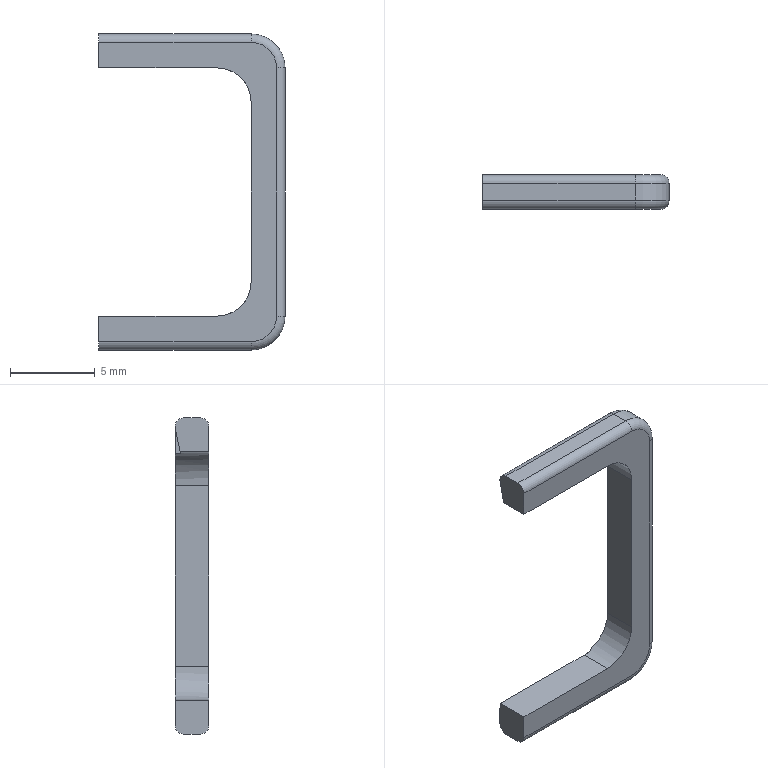Component | SolidWorks | BrushHolder-1 | 1 solid | 30 faces | box 10.95 x 2 x 18.6 mm | volume 140 mm3 | plane 16 | cylinder 10 | torus 4 | commonest cylinder face diameters 1 x6 4 x4
build123d program:
from build123d import *

# Parameters (mm, degrees)
EXTRUDE_THIN1_DEPTH           = 2
FILLET1_R                     = 2
FILLET2_R                     = 0.5
SCOOP_BENDING_CLEARANCE_DEPTH = 7.5


with BuildPart() as part:
    # Sketch1 → Extrude-Thin1 (new body)
    with BuildSketch(Plane.XY):
        Polygon((0, 0), (0, 8.954), (14.597, 8.954), (14.597, 0), (16.597, 0), (16.597, 10.954), (-2, 10.954), (-2, 0), align=None)
    extrude(amount=EXTRUDE_THIN1_DEPTH)

    # Fillet1
    fillet1_edges = [part.edges().sort_by_distance(p)[0] for p in [
        (-2, 10.954, 1),
        (16.597, 10.954, 1),
        (14.597, 8.954, 1),
        (0, 8.954, 1),
    ]]
    fillet(fillet1_edges, radius=FILLET1_R)

    # Fillet2
    fillet2_edges = [part.edges().sort_by_distance(p)[0] for p in [
        (16.597, 4.477, 2),
        (7.298, 10.954, 0),
        (7.298, 10.954, 2),
        (-2, 4.477, 0),
        (-1.414, 10.369, 0),
        (16.011, 10.369, 0),
        (-2, 4.477, 2),
        (-1.414, 10.369, 2),
        (16.011, 10.369, 2),
        (16.597, 4.477, 0),
    ]]
    fillet(fillet2_edges, radius=FILLET2_R)

    # Spatula Clearance Sketch → Scoop Bending Clearance (cut)
    with BuildSketch(Plane.XZ):
        Polygon((-1.456, 0), (0, 0.3), (0.2439, 0.3), (0.2439, -0.2446), (-1.456, -0.2446), align=None)
        Polygon((14.974, 0), (14.597, 0.04539), (14.344, 0.04539), (14.344, -0.2446), (14.974, -0.2446), align=None)
    extrude(amount=-SCOOP_BENDING_CLEARANCE_DEPTH, mode=Mode.SUBTRACT)


solid = part.part

# Placed as in the assembly
solid = solid.moved(Location((-35.654, -76.145, 205.244), (90, 0, -90)))
STEP:
#1=COLOUR_RGB('',0.7922,0.8196,0.9333);
#2=FILL_AREA_STYLE_COLOUR('',#1);
#3=FILL_AREA_STYLE('',(#2));
#4=SURFACE_STYLE_FILL_AREA(#3);
#5=SURFACE_SIDE_STYLE('',(#4));
#6=SURFACE_STYLE_USAGE(.BOTH.,#5);
#7=PRESENTATION_STYLE_ASSIGNMENT((#6));
#8=CARTESIAN_POINT('',(-1.051,-3.057,8.159));
#9=VERTEX_POINT('',#8);
#10=CARTESIAN_POINT('',(-1.051,-3.018,8.159));
#11=VERTEX_POINT('',#10);
#12=CARTESIAN_POINT('',(-1.051,-3.077,8.159));
#13=DIRECTION('',(-0.,1.,-0.));
#14=VECTOR('',#13,39.37);
#15=LINE('',#12,#14);
#16=EDGE_CURVE('',#9,#11,#15,.T.);
#17=ORIENTED_EDGE('',*,*,#16,.T.);
#18=CARTESIAN_POINT('',(-1.404,-3.018,8.159));
#19=VERTEX_POINT('',#18);
#20=CARTESIAN_POINT('',(-1.404,-3.018,8.159));
#21=DIRECTION('',(-1.,-0.,-0.));
#22=VECTOR('',#21,39.37);
#23=LINE('',#20,#22);
#24=EDGE_CURVE('',#11,#19,#23,.T.);
#25=ORIENTED_EDGE('',*,*,#24,.T.);
#26=CARTESIAN_POINT('',(-1.404,-3.057,8.159));
#27=VERTEX_POINT('',#26);
#28=CARTESIAN_POINT('',(-1.404,-3.077,8.159));
#29=DIRECTION('',(-0.,1.,-0.));
#30=VECTOR('',#29,39.37);
#31=LINE('',#28,#30);
#32=EDGE_CURVE('',#27,#19,#31,.T.);
#33=ORIENTED_EDGE('',*,*,#32,.F.);
#34=CARTESIAN_POINT('',(-1.051,-3.057,8.159));
#35=DIRECTION('',(1.,0.,0.));
#36=VECTOR('',#35,39.37);
#37=LINE('',#34,#36);
#38=EDGE_CURVE('',#27,#9,#37,.T.);
#39=ORIENTED_EDGE('',*,*,#38,.T.);
#40=EDGE_LOOP('',(#17,#25,#33,#39));
#41=FACE_OUTER_BOUND('',#40,.T.);
#42=CARTESIAN_POINT('',(-1.404,-3.077,8.159));
#43=DIRECTION('',(0.,-0.,-1.));
#44=DIRECTION('',(-0.,1.,-0.));
#45=AXIS2_PLACEMENT_3D('',#42,#43,#44);
#46=PLANE('',#45);
#47=ADVANCED_FACE('',(#41),#46,.F.);
#48=CARTESIAN_POINT('',(-1.404,-3.01,8.08));
#49=VERTEX_POINT('',#48);
#50=CARTESIAN_POINT('',(-1.404,-2.998,8.138));
#51=VERTEX_POINT('',#50);
#52=CARTESIAN_POINT('',(-1.404,-2.998,8.138));
#53=DIRECTION('',(-0.,0.2018,0.9794));
#54=VECTOR('',#53,39.37);
#55=LINE('',#52,#54);
#56=EDGE_CURVE('',#49,#51,#55,.T.);
#57=ORIENTED_EDGE('',*,*,#56,.F.);
#58=CARTESIAN_POINT('',(-1.404,-3.077,8.08));
#59=VERTEX_POINT('',#58);
#60=CARTESIAN_POINT('',(-1.404,-3.077,8.08));
#61=DIRECTION('',(-0.,1.,-0.));
#62=VECTOR('',#61,39.37);
#63=LINE('',#60,#62);
#64=EDGE_CURVE('',#59,#49,#63,.T.);
#65=ORIENTED_EDGE('',*,*,#64,.F.);
#66=CARTESIAN_POINT('',(-1.404,-3.077,8.14));
#67=VERTEX_POINT('',#66);
#68=CARTESIAN_POINT('',(-1.404,-3.077,8.08));
#69=DIRECTION('',(-0.,0.,1.));
#70=VECTOR('',#69,39.37);
#71=LINE('',#68,#70);
#72=EDGE_CURVE('',#59,#67,#71,.T.);
#73=ORIENTED_EDGE('',*,*,#72,.T.);
#74=CARTESIAN_POINT('',(-1.404,-3.057,8.14));
#75=DIRECTION('',(-1.,-0.,-0.));
#76=DIRECTION('',(0.,1.,0.));
#77=AXIS2_PLACEMENT_3D('',#74,#75,#76);
#78=CIRCLE('',#77,0.01969);
#79=EDGE_CURVE('',#67,#27,#78,.T.);
#80=ORIENTED_EDGE('',*,*,#79,.T.);
#81=ORIENTED_EDGE('',*,*,#32,.T.);
#82=CARTESIAN_POINT('',(-1.404,-2.998,8.14));
#83=VERTEX_POINT('',#82);
#84=CARTESIAN_POINT('',(-1.404,-3.018,8.14));
#85=DIRECTION('',(-1.,-0.,-0.));
#86=DIRECTION('',(0.,1.,0.));
#87=AXIS2_PLACEMENT_3D('',#84,#85,#86);
#88=CIRCLE('',#87,0.01969);
#89=EDGE_CURVE('',#19,#83,#88,.T.);
#90=ORIENTED_EDGE('',*,*,#89,.T.);
#91=CARTESIAN_POINT('',(-1.404,-2.998,8.08));
#92=DIRECTION('',(-0.,0.,1.));
#93=VECTOR('',#92,39.37);
#94=LINE('',#91,#93);
#95=EDGE_CURVE('',#51,#83,#94,.T.);
#96=ORIENTED_EDGE('',*,*,#95,.F.);
#97=EDGE_LOOP('',(#57,#65,#73,#80,#81,#90,#96));
#98=FACE_OUTER_BOUND('',#97,.T.);
#99=CARTESIAN_POINT('',(-1.404,-3.077,8.08));
#100=DIRECTION('',(-1.,-0.,-0.));
#101=DIRECTION('',(-0.,1.,-0.));
#102=AXIS2_PLACEMENT_3D('',#99,#100,#101);
#103=PLANE('',#102);
#104=ADVANCED_FACE('',(#98),#103,.T.);
#105=CARTESIAN_POINT('',(-1.13,-3.01,8.08));
#106=VERTEX_POINT('',#105);
#107=CARTESIAN_POINT('',(-1.108,-3.01,8.08));
#108=DIRECTION('',(-1.,-0.,-0.));
#109=VECTOR('',#108,39.37);
#110=LINE('',#107,#109);
#111=EDGE_CURVE('',#106,#49,#110,.T.);
#112=ORIENTED_EDGE('',*,*,#111,.F.);
#113=CARTESIAN_POINT('',(-1.13,-3.077,8.08));
#114=VERTEX_POINT('',#113);
#115=CARTESIAN_POINT('',(-1.13,-3.077,8.08));
#116=DIRECTION('',(0.,-1.,0.));
#117=VECTOR('',#116,39.37);
#118=LINE('',#115,#117);
#119=EDGE_CURVE('',#106,#114,#118,.T.);
#120=ORIENTED_EDGE('',*,*,#119,.T.);
#121=CARTESIAN_POINT('',(-1.404,-3.077,8.08));
#122=DIRECTION('',(-1.,-0.,-0.));
#123=VECTOR('',#122,39.37);
#124=LINE('',#121,#123);
#125=EDGE_CURVE('',#114,#59,#124,.T.);
#126=ORIENTED_EDGE('',*,*,#125,.T.);
#127=ORIENTED_EDGE('',*,*,#64,.T.);
#128=EDGE_LOOP('',(#112,#120,#126,#127));
#129=FACE_OUTER_BOUND('',#128,.T.);
#130=CARTESIAN_POINT('',(-1.404,-3.077,8.08));
#131=DIRECTION('',(0.,-0.,-1.));
#132=DIRECTION('',(-0.,1.,-0.));
#133=AXIS2_PLACEMENT_3D('',#130,#131,#132);
#134=PLANE('',#133);
#135=ADVANCED_FACE('',(#129),#134,.T.);
#136=CARTESIAN_POINT('',(-1.051,-2.998,7.585));
#137=VERTEX_POINT('',#136);
#138=CARTESIAN_POINT('',(-1.051,-2.998,8.002));
#139=VERTEX_POINT('',#138);
#140=CARTESIAN_POINT('',(-1.051,-2.998,8.08));
#141=DIRECTION('',(-0.,0.,1.));
#142=VECTOR('',#141,39.37);
#143=LINE('',#140,#142);
#144=EDGE_CURVE('',#137,#139,#143,.T.);
#145=ORIENTED_EDGE('',*,*,#144,.F.);
#146=CARTESIAN_POINT('',(-1.051,-3.077,7.585));
#147=VERTEX_POINT('',#146);
#148=CARTESIAN_POINT('',(-1.051,-3.077,7.585));
#149=DIRECTION('',(0.,-1.,0.));
#150=VECTOR('',#149,39.37);
#151=LINE('',#148,#150);
#152=EDGE_CURVE('',#137,#147,#151,.T.);
#153=ORIENTED_EDGE('',*,*,#152,.T.);
#154=CARTESIAN_POINT('',(-1.051,-3.077,8.002));
#155=VERTEX_POINT('',#154);
#156=CARTESIAN_POINT('',(-1.051,-3.077,8.08));
#157=DIRECTION('',(-0.,0.,1.));
#158=VECTOR('',#157,39.37);
#159=LINE('',#156,#158);
#160=EDGE_CURVE('',#147,#155,#159,.T.);
#161=ORIENTED_EDGE('',*,*,#160,.T.);
#162=CARTESIAN_POINT('',(-1.051,-2.998,8.002));
#163=DIRECTION('',(-0.,1.,-0.));
#164=VECTOR('',#163,39.37);
#165=LINE('',#162,#164);
#166=EDGE_CURVE('',#155,#139,#165,.T.);
#167=ORIENTED_EDGE('',*,*,#166,.T.);
#168=EDGE_LOOP('',(#145,#153,#161,#167));
#169=FACE_OUTER_BOUND('',#168,.T.);
#170=CARTESIAN_POINT('',(-1.051,-3.077,8.08));
#171=DIRECTION('',(-1.,-0.,-0.));
#172=DIRECTION('',(-0.,1.,-0.));
#173=AXIS2_PLACEMENT_3D('',#170,#171,#172);
#174=PLANE('',#173);
#175=ADVANCED_FACE('',(#169),#174,.T.);
#176=CARTESIAN_POINT('',(-1.13,-3.,7.506));
#177=VERTEX_POINT('',#176);
#178=CARTESIAN_POINT('',(-1.404,-3.,7.506));
#179=VERTEX_POINT('',#178);
#180=CARTESIAN_POINT('',(-1.108,-3.,7.506));
#181=DIRECTION('',(-1.,-0.,-0.));
#182=VECTOR('',#181,39.37);
#183=LINE('',#180,#182);
#184=EDGE_CURVE('',#177,#179,#183,.T.);
#185=ORIENTED_EDGE('',*,*,#184,.T.);
#186=CARTESIAN_POINT('',(-1.404,-3.077,7.506));
#187=VERTEX_POINT('',#186);
#188=CARTESIAN_POINT('',(-1.404,-3.077,7.506));
#189=DIRECTION('',(-0.,1.,-0.));
#190=VECTOR('',#189,39.37);
#191=LINE('',#188,#190);
#192=EDGE_CURVE('',#187,#179,#191,.T.);
#193=ORIENTED_EDGE('',*,*,#192,.F.);
#194=CARTESIAN_POINT('',(-1.13,-3.077,7.506));
#195=VERTEX_POINT('',#194);
#196=CARTESIAN_POINT('',(-1.404,-3.077,7.506));
#197=DIRECTION('',(1.,0.,0.));
#198=VECTOR('',#197,39.37);
#199=LINE('',#196,#198);
#200=EDGE_CURVE('',#187,#195,#199,.T.);
#201=ORIENTED_EDGE('',*,*,#200,.T.);
#202=CARTESIAN_POINT('',(-1.13,-2.998,7.506));
#203=DIRECTION('',(-0.,1.,-0.));
#204=VECTOR('',#203,39.37);
#205=LINE('',#202,#204);
#206=EDGE_CURVE('',#195,#177,#205,.T.);
#207=ORIENTED_EDGE('',*,*,#206,.T.);
#208=EDGE_LOOP('',(#185,#193,#201,#207));
#209=FACE_OUTER_BOUND('',#208,.T.);
#210=CARTESIAN_POINT('',(-1.404,-3.077,7.506));
#211=DIRECTION('',(-0.,0.,1.));
#212=DIRECTION('',(0.,-1.,0.));
#213=AXIS2_PLACEMENT_3D('',#210,#211,#212);
#214=PLANE('',#213);
#215=ADVANCED_FACE('',(#209),#214,.T.);
#216=CARTESIAN_POINT('',(-1.404,-2.998,7.491));
#217=VERTEX_POINT('',#216);
#218=CARTESIAN_POINT('',(-1.404,-2.998,7.491));
#219=DIRECTION('',(-0.,-0.1195,0.9928));
#220=VECTOR('',#219,39.37);
#221=LINE('',#218,#220);
#222=EDGE_CURVE('',#217,#179,#221,.T.);
#223=ORIENTED_EDGE('',*,*,#222,.F.);
#224=CARTESIAN_POINT('',(-1.404,-2.998,7.447));
#225=VERTEX_POINT('',#224);
#226=CARTESIAN_POINT('',(-1.404,-2.998,7.427));
#227=DIRECTION('',(-0.,0.,1.));
#228=VECTOR('',#227,39.37);
#229=LINE('',#226,#228);
#230=EDGE_CURVE('',#225,#217,#229,.T.);
#231=ORIENTED_EDGE('',*,*,#230,.F.);
#232=CARTESIAN_POINT('',(-1.404,-3.018,7.427));
#233=VERTEX_POINT('',#232);
#234=CARTESIAN_POINT('',(-1.404,-3.018,7.447));
#235=DIRECTION('',(-1.,-0.,-0.));
#236=DIRECTION('',(0.,1.,0.));
#237=AXIS2_PLACEMENT_3D('',#234,#235,#236);
#238=CIRCLE('',#237,0.01969);
#239=EDGE_CURVE('',#225,#233,#238,.T.);
#240=ORIENTED_EDGE('',*,*,#239,.T.);
#241=CARTESIAN_POINT('',(-1.404,-3.057,7.427));
#242=VERTEX_POINT('',#241);
#243=CARTESIAN_POINT('',(-1.404,-3.077,7.427));
#244=DIRECTION('',(-0.,1.,-0.));
#245=VECTOR('',#244,39.37);
#246=LINE('',#243,#245);
#247=EDGE_CURVE('',#242,#233,#246,.T.);
#248=ORIENTED_EDGE('',*,*,#247,.F.);
#249=CARTESIAN_POINT('',(-1.404,-3.077,7.447));
#250=VERTEX_POINT('',#249);
#251=CARTESIAN_POINT('',(-1.404,-3.057,7.447));
#252=DIRECTION('',(-1.,-0.,-0.));
#253=DIRECTION('',(0.,1.,0.));
#254=AXIS2_PLACEMENT_3D('',#251,#252,#253);
#255=CIRCLE('',#254,0.01969);
#256=EDGE_CURVE('',#242,#250,#255,.T.);
#257=ORIENTED_EDGE('',*,*,#256,.T.);
#258=CARTESIAN_POINT('',(-1.404,-3.077,7.427));
#259=DIRECTION('',(-0.,0.,1.));
#260=VECTOR('',#259,39.37);
#261=LINE('',#258,#260);
#262=EDGE_CURVE('',#250,#187,#261,.T.);
#263=ORIENTED_EDGE('',*,*,#262,.T.);
#264=ORIENTED_EDGE('',*,*,#192,.T.);
#265=EDGE_LOOP('',(#223,#231,#240,#248,#257,#263,#264));
#266=FACE_OUTER_BOUND('',#265,.T.);
#267=CARTESIAN_POINT('',(-1.404,-3.077,7.427));
#268=DIRECTION('',(-1.,-0.,-0.));
#269=DIRECTION('',(-0.,1.,-0.));
#270=AXIS2_PLACEMENT_3D('',#267,#268,#269);
#271=PLANE('',#270);
#272=ADVANCED_FACE('',(#266),#271,.T.);
#273=ORIENTED_EDGE('',*,*,#247,.T.);
#274=CARTESIAN_POINT('',(-1.051,-3.018,7.427));
#275=VERTEX_POINT('',#274);
#276=CARTESIAN_POINT('',(-1.404,-3.018,7.427));
#277=DIRECTION('',(1.,0.,0.));
#278=VECTOR('',#277,39.37);
#279=LINE('',#276,#278);
#280=EDGE_CURVE('',#233,#275,#279,.T.);
#281=ORIENTED_EDGE('',*,*,#280,.T.);
#282=CARTESIAN_POINT('',(-1.051,-3.057,7.427));
#283=VERTEX_POINT('',#282);
#284=CARTESIAN_POINT('',(-1.051,-3.077,7.427));
#285=DIRECTION('',(0.,-1.,0.));
#286=VECTOR('',#285,39.37);
#287=LINE('',#284,#286);
#288=EDGE_CURVE('',#275,#283,#287,.T.);
#289=ORIENTED_EDGE('',*,*,#288,.T.);
#290=CARTESIAN_POINT('',(-1.404,-3.057,7.427));
#291=DIRECTION('',(-1.,-0.,-0.));
#292=VECTOR('',#291,39.37);
#293=LINE('',#290,#292);
#294=EDGE_CURVE('',#283,#242,#293,.T.);
#295=ORIENTED_EDGE('',*,*,#294,.T.);
#296=EDGE_LOOP('',(#273,#281,#289,#295));
#297=FACE_OUTER_BOUND('',#296,.T.);
#298=CARTESIAN_POINT('',(-1.404,-3.077,7.427));
#299=DIRECTION('',(-0.,0.,1.));
#300=DIRECTION('',(0.,-1.,0.));
#301=AXIS2_PLACEMENT_3D('',#298,#299,#300);
#302=PLANE('',#301);
#303=ADVANCED_FACE('',(#297),#302,.F.);
#304=CARTESIAN_POINT('',(-0.9724,-3.057,7.506));
#305=VERTEX_POINT('',#304);
#306=CARTESIAN_POINT('',(-0.9724,-3.018,7.506));
#307=VERTEX_POINT('',#306);
#308=CARTESIAN_POINT('',(-0.9724,-3.077,7.506));
#309=DIRECTION('',(-0.,1.,-0.));
#310=VECTOR('',#309,39.37);
#311=LINE('',#308,#310);
#312=EDGE_CURVE('',#305,#307,#311,.T.);
#313=ORIENTED_EDGE('',*,*,#312,.T.);
#314=CARTESIAN_POINT('',(-0.9724,-3.018,8.08));
#315=VERTEX_POINT('',#314);
#316=CARTESIAN_POINT('',(-0.9724,-3.018,8.08));
#317=DIRECTION('',(-0.,0.,1.));
#318=VECTOR('',#317,39.37);
#319=LINE('',#316,#318);
#320=EDGE_CURVE('',#307,#315,#319,.T.);
#321=ORIENTED_EDGE('',*,*,#320,.T.);
#322=CARTESIAN_POINT('',(-0.9724,-3.057,8.08));
#323=VERTEX_POINT('',#322);
#324=CARTESIAN_POINT('',(-0.9724,-3.077,8.08));
#325=DIRECTION('',(0.,-1.,0.));
#326=VECTOR('',#325,39.37);
#327=LINE('',#324,#326);
#328=EDGE_CURVE('',#315,#323,#327,.T.);
#329=ORIENTED_EDGE('',*,*,#328,.T.);
#330=CARTESIAN_POINT('',(-0.9724,-3.057,7.506));
#331=DIRECTION('',(0.,-0.,-1.));
#332=VECTOR('',#331,39.37);
#333=LINE('',#330,#332);
#334=EDGE_CURVE('',#323,#305,#333,.T.);
#335=ORIENTED_EDGE('',*,*,#334,.T.);
#336=EDGE_LOOP('',(#313,#321,#329,#335));
#337=FACE_OUTER_BOUND('',#336,.T.);
#338=CARTESIAN_POINT('',(-0.9724,-3.077,8.08));
#339=DIRECTION('',(-1.,-0.,-0.));
#340=DIRECTION('',(-0.,1.,-0.));
#341=AXIS2_PLACEMENT_3D('',#338,#339,#340);
#342=PLANE('',#341);
#343=ADVANCED_FACE('',(#337),#342,.F.);
#344=ORIENTED_EDGE('',*,*,#262,.F.);
#345=CARTESIAN_POINT('',(-1.051,-3.077,7.447));
#346=VERTEX_POINT('',#345);
#347=CARTESIAN_POINT('',(-1.051,-3.077,7.447));
#348=DIRECTION('',(1.,0.,0.));
#349=VECTOR('',#348,39.37);
#350=LINE('',#347,#349);
#351=EDGE_CURVE('',#250,#346,#350,.T.);
#352=ORIENTED_EDGE('',*,*,#351,.T.);
#353=CARTESIAN_POINT('',(-0.9921,-3.077,7.506));
#354=VERTEX_POINT('',#353);
#355=CARTESIAN_POINT('',(-1.051,-3.077,7.506));
#356=DIRECTION('',(0.,-1.,0.));
#357=DIRECTION('',(0.,0.,-1.));
#358=AXIS2_PLACEMENT_3D('',#355,#356,#357);
#359=CIRCLE('',#358,0.05906);
#360=EDGE_CURVE('',#346,#354,#359,.T.);
#361=ORIENTED_EDGE('',*,*,#360,.T.);
#362=CARTESIAN_POINT('',(-0.9921,-3.077,8.08));
#363=VERTEX_POINT('',#362);
#364=CARTESIAN_POINT('',(-0.9921,-3.077,8.08));
#365=DIRECTION('',(-0.,0.,1.));
#366=VECTOR('',#365,39.37);
#367=LINE('',#364,#366);
#368=EDGE_CURVE('',#354,#363,#367,.T.);
#369=ORIENTED_EDGE('',*,*,#368,.T.);
#370=CARTESIAN_POINT('',(-1.051,-3.077,8.14));
#371=VERTEX_POINT('',#370);
#372=CARTESIAN_POINT('',(-1.051,-3.077,8.08));
#373=DIRECTION('',(0.,-1.,0.));
#374=DIRECTION('',(0.,0.,-1.));
#375=AXIS2_PLACEMENT_3D('',#372,#373,#374);
#376=CIRCLE('',#375,0.05906);
#377=EDGE_CURVE('',#363,#371,#376,.T.);
#378=ORIENTED_EDGE('',*,*,#377,.T.);
#379=CARTESIAN_POINT('',(-1.404,-3.077,8.14));
#380=DIRECTION('',(-1.,-0.,-0.));
#381=VECTOR('',#380,39.37);
#382=LINE('',#379,#381);
#383=EDGE_CURVE('',#371,#67,#382,.T.);
#384=ORIENTED_EDGE('',*,*,#383,.T.);
#385=ORIENTED_EDGE('',*,*,#72,.F.);
#386=ORIENTED_EDGE('',*,*,#125,.F.);
#387=CARTESIAN_POINT('',(-1.13,-3.077,8.002));
#388=DIRECTION('',(-0.,1.,-0.));
#389=DIRECTION('',(0.,0.,-1.));
#390=AXIS2_PLACEMENT_3D('',#387,#388,#389);
#391=CIRCLE('',#390,0.07874);
#392=EDGE_CURVE('',#114,#155,#391,.T.);
#393=ORIENTED_EDGE('',*,*,#392,.T.);
#394=ORIENTED_EDGE('',*,*,#160,.F.);
#395=CARTESIAN_POINT('',(-1.13,-3.077,7.585));
#396=DIRECTION('',(-0.,1.,-0.));
#397=DIRECTION('',(0.,0.,-1.));
#398=AXIS2_PLACEMENT_3D('',#395,#396,#397);
#399=CIRCLE('',#398,0.07874);
#400=EDGE_CURVE('',#147,#195,#399,.T.);
#401=ORIENTED_EDGE('',*,*,#400,.T.);
#402=ORIENTED_EDGE('',*,*,#200,.F.);
#403=EDGE_LOOP('',(#344,#352,#361,#369,#378,#384,#385,#386,#393,#394,#401,#402));
#404=FACE_OUTER_BOUND('',#403,.T.);
#405=CARTESIAN_POINT('',(-1.404,-3.077,8.08));
#406=DIRECTION('',(0.,-1.,0.));
#407=DIRECTION('',(0.,-0.,-1.));
#408=AXIS2_PLACEMENT_3D('',#405,#406,#407);
#409=PLANE('',#408);
#410=ADVANCED_FACE('',(#404),#409,.T.);
#411=CARTESIAN_POINT('',(-1.108,-2.998,8.077));
#412=VERTEX_POINT('',#411);
#413=CARTESIAN_POINT('',(-1.108,-2.998,8.138));
#414=VERTEX_POINT('',#413);
#415=CARTESIAN_POINT('',(-1.108,-2.998,8.08));
#416=DIRECTION('',(-0.,0.,1.));
#417=VECTOR('',#416,39.37);
#418=LINE('',#415,#417);
#419=EDGE_CURVE('',#412,#414,#418,.T.);
#420=ORIENTED_EDGE('',*,*,#419,.T.);
#421=CARTESIAN_POINT('',(-1.108,-2.998,8.138));
#422=DIRECTION('',(-1.,-0.,-0.));
#423=VECTOR('',#422,39.37);
#424=LINE('',#421,#423);
#425=EDGE_CURVE('',#414,#51,#424,.T.);
#426=ORIENTED_EDGE('',*,*,#425,.T.);
#427=ORIENTED_EDGE('',*,*,#95,.T.);
#428=CARTESIAN_POINT('',(-1.051,-2.998,8.14));
#429=VERTEX_POINT('',#428);
#430=CARTESIAN_POINT('',(-1.404,-2.998,8.14));
#431=DIRECTION('',(1.,0.,0.));
#432=VECTOR('',#431,39.37);
#433=LINE('',#430,#432);
#434=EDGE_CURVE('',#83,#429,#433,.T.);
#435=ORIENTED_EDGE('',*,*,#434,.T.);
#436=CARTESIAN_POINT('',(-0.9921,-2.998,8.08));
#437=VERTEX_POINT('',#436);
#438=CARTESIAN_POINT('',(-1.051,-2.998,8.08));
#439=DIRECTION('',(-0.,1.,-0.));
#440=DIRECTION('',(0.,0.,-1.));
#441=AXIS2_PLACEMENT_3D('',#438,#439,#440);
#442=CIRCLE('',#441,0.05906);
#443=EDGE_CURVE('',#429,#437,#442,.T.);
#444=ORIENTED_EDGE('',*,*,#443,.T.);
#445=CARTESIAN_POINT('',(-0.9921,-2.998,7.506));
#446=VERTEX_POINT('',#445);
#447=CARTESIAN_POINT('',(-0.9921,-2.998,8.08));
#448=DIRECTION('',(0.,-0.,-1.));
#449=VECTOR('',#448,39.37);
#450=LINE('',#447,#449);
#451=EDGE_CURVE('',#437,#446,#450,.T.);
#452=ORIENTED_EDGE('',*,*,#451,.T.);
#453=CARTESIAN_POINT('',(-1.051,-2.998,7.447));
#454=VERTEX_POINT('',#453);
#455=CARTESIAN_POINT('',(-1.051,-2.998,7.506));
#456=DIRECTION('',(-0.,1.,-0.));
#457=DIRECTION('',(0.,0.,-1.));
#458=AXIS2_PLACEMENT_3D('',#455,#456,#457);
#459=CIRCLE('',#458,0.05906);
#460=EDGE_CURVE('',#446,#454,#459,.T.);
#461=ORIENTED_EDGE('',*,*,#460,.T.);
#462=CARTESIAN_POINT('',(-1.404,-2.998,7.447));
#463=DIRECTION('',(-1.,-0.,-0.));
#464=VECTOR('',#463,39.37);
#465=LINE('',#462,#464);
#466=EDGE_CURVE('',#454,#225,#465,.T.);
#467=ORIENTED_EDGE('',*,*,#466,.T.);
#468=ORIENTED_EDGE('',*,*,#230,.T.);
#469=CARTESIAN_POINT('',(-1.108,-2.998,7.491));
#470=VERTEX_POINT('',#469);
#471=CARTESIAN_POINT('',(-1.108,-2.998,7.491));
#472=DIRECTION('',(-1.,-0.,-0.));
#473=VECTOR('',#472,39.37);
#474=LINE('',#471,#473);
#475=EDGE_CURVE('',#470,#217,#474,.T.);
#476=ORIENTED_EDGE('',*,*,#475,.F.);
#477=CARTESIAN_POINT('',(-1.108,-2.998,7.509));
#478=VERTEX_POINT('',#477);
#479=CARTESIAN_POINT('',(-1.108,-2.998,8.08));
#480=DIRECTION('',(0.,-0.,-1.));
#481=VECTOR('',#480,39.37);
#482=LINE('',#479,#481);
#483=EDGE_CURVE('',#478,#470,#482,.T.);
#484=ORIENTED_EDGE('',*,*,#483,.F.);
#485=CARTESIAN_POINT('',(-1.13,-2.998,7.585));
#486=DIRECTION('',(0.,-1.,0.));
#487=DIRECTION('',(0.,0.,-1.));
#488=AXIS2_PLACEMENT_3D('',#485,#486,#487);
#489=CIRCLE('',#488,0.07874);
#490=EDGE_CURVE('',#478,#137,#489,.T.);
#491=ORIENTED_EDGE('',*,*,#490,.T.);
#492=ORIENTED_EDGE('',*,*,#144,.T.);
#493=CARTESIAN_POINT('',(-1.13,-2.998,8.002));
#494=DIRECTION('',(0.,-1.,0.));
#495=DIRECTION('',(0.,0.,-1.));
#496=AXIS2_PLACEMENT_3D('',#493,#494,#495);
#497=CIRCLE('',#496,0.07874);
#498=EDGE_CURVE('',#139,#412,#497,.T.);
#499=ORIENTED_EDGE('',*,*,#498,.T.);
#500=EDGE_LOOP('',(#420,#426,#427,#435,#444,#452,#461,#467,#468,#476,#484,#491,#492,#499));
#501=FACE_OUTER_BOUND('',#500,.T.);
#502=CARTESIAN_POINT('',(-1.404,-2.998,8.08));
#503=DIRECTION('',(0.,-1.,0.));
#504=DIRECTION('',(0.,-0.,-1.));
#505=AXIS2_PLACEMENT_3D('',#502,#503,#504);
#506=PLANE('',#505);
#507=ADVANCED_FACE('',(#501),#506,.F.);
#508=CARTESIAN_POINT('',(-1.108,-3.,7.509));
#509=VERTEX_POINT('',#508);
#510=CARTESIAN_POINT('',(-1.108,-3.077,7.509));
#511=DIRECTION('',(-0.,1.,-0.));
#512=VECTOR('',#511,39.37);
#513=LINE('',#510,#512);
#514=EDGE_CURVE('',#509,#478,#513,.T.);
#515=ORIENTED_EDGE('',*,*,#514,.F.);
#516=CARTESIAN_POINT('',(-1.13,-3.,7.585));
#517=DIRECTION('',(-0.,1.,-0.));
#518=DIRECTION('',(0.,0.,-1.));
#519=AXIS2_PLACEMENT_3D('',#516,#517,#518);
#520=CIRCLE('',#519,0.07874);
#521=EDGE_CURVE('',#509,#177,#520,.T.);
#522=ORIENTED_EDGE('',*,*,#521,.T.);
#523=ORIENTED_EDGE('',*,*,#206,.F.);
#524=ORIENTED_EDGE('',*,*,#400,.F.);
#525=ORIENTED_EDGE('',*,*,#152,.F.);
#526=ORIENTED_EDGE('',*,*,#490,.F.);
#527=EDGE_LOOP('',(#515,#522,#523,#524,#525,#526));
#528=FACE_OUTER_BOUND('',#527,.T.);
#529=CARTESIAN_POINT('',(-1.13,-3.077,7.585));
#530=DIRECTION('',(0.,-1.,0.));
#531=DIRECTION('',(0.,0.,-1.));
#532=AXIS2_PLACEMENT_3D('',#529,#530,#531);
#533=CYLINDRICAL_SURFACE('',#532,0.07874);
#534=ADVANCED_FACE('',(#528),#533,.F.);
#535=ORIENTED_EDGE('',*,*,#119,.F.);
#536=CARTESIAN_POINT('',(-1.108,-3.01,8.077));
#537=VERTEX_POINT('',#536);
#538=CARTESIAN_POINT('',(-1.13,-3.01,8.002));
#539=DIRECTION('',(-0.,1.,-0.));
#540=DIRECTION('',(0.,0.,-1.));
#541=AXIS2_PLACEMENT_3D('',#538,#539,#540);
#542=CIRCLE('',#541,0.07874);
#543=EDGE_CURVE('',#106,#537,#542,.T.);
#544=ORIENTED_EDGE('',*,*,#543,.T.);
#545=CARTESIAN_POINT('',(-1.108,-3.077,8.077));
#546=DIRECTION('',(-0.,1.,-0.));
#547=VECTOR('',#546,39.37);
#548=LINE('',#545,#547);
#549=EDGE_CURVE('',#537,#412,#548,.T.);
#550=ORIENTED_EDGE('',*,*,#549,.T.);
#551=ORIENTED_EDGE('',*,*,#498,.F.);
#552=ORIENTED_EDGE('',*,*,#166,.F.);
#553=ORIENTED_EDGE('',*,*,#392,.F.);
#554=EDGE_LOOP('',(#535,#544,#550,#551,#552,#553));
#555=FACE_OUTER_BOUND('',#554,.T.);
#556=CARTESIAN_POINT('',(-1.13,-3.077,8.002));
#557=DIRECTION('',(0.,-1.,0.));
#558=DIRECTION('',(0.,0.,-1.));
#559=AXIS2_PLACEMENT_3D('',#556,#557,#558);
#560=CYLINDRICAL_SURFACE('',#559,0.07874);
#561=ADVANCED_FACE('',(#555),#560,.F.);
#562=ORIENTED_EDGE('',*,*,#288,.F.);
#563=CARTESIAN_POINT('',(-1.051,-3.018,7.506));
#564=DIRECTION('',(0.,-1.,0.));
#565=DIRECTION('',(0.,0.,-1.));
#566=AXIS2_PLACEMENT_3D('',#563,#564,#565);
#567=CIRCLE('',#566,0.07874);
#568=EDGE_CURVE('',#275,#307,#567,.T.);
#569=ORIENTED_EDGE('',*,*,#568,.T.);
#570=ORIENTED_EDGE('',*,*,#312,.F.);
#571=CARTESIAN_POINT('',(-1.051,-3.057,7.506));
#572=DIRECTION('',(-0.,1.,-0.));
#573=DIRECTION('',(0.,0.,-1.));
#574=AXIS2_PLACEMENT_3D('',#571,#572,#573);
#575=CIRCLE('',#574,0.07874);
#576=EDGE_CURVE('',#305,#283,#575,.T.);
#577=ORIENTED_EDGE('',*,*,#576,.T.);
#578=EDGE_LOOP('',(#562,#569,#570,#577));
#579=FACE_OUTER_BOUND('',#578,.T.);
#580=CARTESIAN_POINT('',(-1.051,-3.077,7.506));
#581=DIRECTION('',(-0.,1.,-0.));
#582=DIRECTION('',(0.,0.,1.));
#583=AXIS2_PLACEMENT_3D('',#580,#581,#582);
#584=CYLINDRICAL_SURFACE('',#583,0.07874);
#585=ADVANCED_FACE('',(#579),#584,.T.);
#586=ORIENTED_EDGE('',*,*,#328,.F.);
#587=CARTESIAN_POINT('',(-1.051,-3.018,8.08));
#588=DIRECTION('',(0.,-1.,0.));
#589=DIRECTION('',(0.,0.,-1.));
#590=AXIS2_PLACEMENT_3D('',#587,#588,#589);
#591=CIRCLE('',#590,0.07874);
#592=EDGE_CURVE('',#315,#11,#591,.T.);
#593=ORIENTED_EDGE('',*,*,#592,.T.);
#594=ORIENTED_EDGE('',*,*,#16,.F.);
#595=CARTESIAN_POINT('',(-1.051,-3.057,8.08));
#596=DIRECTION('',(-0.,1.,-0.));
#597=DIRECTION('',(0.,0.,-1.));
#598=AXIS2_PLACEMENT_3D('',#595,#596,#597);
#599=CIRCLE('',#598,0.07874);
#600=EDGE_CURVE('',#9,#323,#599,.T.);
#601=ORIENTED_EDGE('',*,*,#600,.T.);
#602=EDGE_LOOP('',(#586,#593,#594,#601));
#603=FACE_OUTER_BOUND('',#602,.T.);
#604=CARTESIAN_POINT('',(-1.051,-3.077,8.08));
#605=DIRECTION('',(-0.,1.,-0.));
#606=DIRECTION('',(0.,0.,1.));
#607=AXIS2_PLACEMENT_3D('',#604,#605,#606);
#608=CYLINDRICAL_SURFACE('',#607,0.07874);
#609=ADVANCED_FACE('',(#603),#608,.T.);
#610=ORIENTED_EDGE('',*,*,#89,.F.);
#611=ORIENTED_EDGE('',*,*,#24,.F.);
#612=CARTESIAN_POINT('',(-1.051,-3.018,8.14));
#613=DIRECTION('',(1.,0.,0.));
#614=DIRECTION('',(0.,-1.,0.));
#615=AXIS2_PLACEMENT_3D('',#612,#613,#614);
#616=CIRCLE('',#615,0.01969);
#617=EDGE_CURVE('',#429,#11,#616,.T.);
#618=ORIENTED_EDGE('',*,*,#617,.F.);
#619=ORIENTED_EDGE('',*,*,#434,.F.);
#620=EDGE_LOOP('',(#610,#611,#618,#619));
#621=FACE_OUTER_BOUND('',#620,.T.);
#622=CARTESIAN_POINT('',(-1.404,-3.018,8.14));
#623=DIRECTION('',(-1.,-0.,-0.));
#624=DIRECTION('',(0.,1.,0.));
#625=AXIS2_PLACEMENT_3D('',#622,#623,#624);
#626=CYLINDRICAL_SURFACE('',#625,0.01969);
#627=ADVANCED_FACE('',(#621),#626,.T.);
#628=ORIENTED_EDGE('',*,*,#617,.T.);
#629=ORIENTED_EDGE('',*,*,#592,.F.);
#630=CARTESIAN_POINT('',(-0.9921,-3.018,8.08));
#631=DIRECTION('',(0.,-0.,-1.));
#632=DIRECTION('',(0.,1.,0.));
#633=AXIS2_PLACEMENT_3D('',#630,#631,#632);
#634=CIRCLE('',#633,0.01969);
#635=EDGE_CURVE('',#437,#315,#634,.T.);
#636=ORIENTED_EDGE('',*,*,#635,.F.);
#637=ORIENTED_EDGE('',*,*,#443,.F.);
#638=EDGE_LOOP('',(#628,#629,#636,#637));
#639=FACE_OUTER_BOUND('',#638,.T.);
#640=CARTESIAN_POINT('',(-1.051,-3.018,8.08));
#641=DIRECTION('',(0.,-1.,0.));
#642=DIRECTION('',(0.,-0.,-1.));
#643=AXIS2_PLACEMENT_3D('',#640,#641,#642);
#644=TOROIDAL_SURFACE('',#643,0.05906,0.01969);
#645=ADVANCED_FACE('',(#639),#644,.T.);
#646=ORIENTED_EDGE('',*,*,#635,.T.);
#647=ORIENTED_EDGE('',*,*,#320,.F.);
#648=CARTESIAN_POINT('',(-0.9921,-3.018,7.506));
#649=DIRECTION('',(0.,-0.,-1.));
#650=DIRECTION('',(0.,1.,0.));
#651=AXIS2_PLACEMENT_3D('',#648,#649,#650);
#652=CIRCLE('',#651,0.01969);
#653=EDGE_CURVE('',#446,#307,#652,.T.);
#654=ORIENTED_EDGE('',*,*,#653,.F.);
#655=ORIENTED_EDGE('',*,*,#451,.F.);
#656=EDGE_LOOP('',(#646,#647,#654,#655));
#657=FACE_OUTER_BOUND('',#656,.T.);
#658=CARTESIAN_POINT('',(-0.9921,-3.018,8.08));
#659=DIRECTION('',(-0.,0.,1.));
#660=DIRECTION('',(0.,-1.,0.));
#661=AXIS2_PLACEMENT_3D('',#658,#659,#660);
#662=CYLINDRICAL_SURFACE('',#661,0.01969);
#663=ADVANCED_FACE('',(#657),#662,.T.);
#664=ORIENTED_EDGE('',*,*,#653,.T.);
#665=ORIENTED_EDGE('',*,*,#568,.F.);
#666=CARTESIAN_POINT('',(-1.051,-3.018,7.447));
#667=DIRECTION('',(-1.,-0.,-0.));
#668=DIRECTION('',(0.,1.,0.));
#669=AXIS2_PLACEMENT_3D('',#666,#667,#668);
#670=CIRCLE('',#669,0.01969);
#671=EDGE_CURVE('',#454,#275,#670,.T.);
#672=ORIENTED_EDGE('',*,*,#671,.F.);
#673=ORIENTED_EDGE('',*,*,#460,.F.);
#674=EDGE_LOOP('',(#664,#665,#672,#673));
#675=FACE_OUTER_BOUND('',#674,.T.);
#676=CARTESIAN_POINT('',(-1.051,-3.018,7.506));
#677=DIRECTION('',(0.,-1.,0.));
#678=DIRECTION('',(0.,-0.,-1.));
#679=AXIS2_PLACEMENT_3D('',#676,#677,#678);
#680=TOROIDAL_SURFACE('',#679,0.05906,0.01969);
#681=ADVANCED_FACE('',(#675),#680,.T.);
#682=ORIENTED_EDGE('',*,*,#239,.F.);
#683=ORIENTED_EDGE('',*,*,#466,.F.);
#684=ORIENTED_EDGE('',*,*,#671,.T.);
#685=ORIENTED_EDGE('',*,*,#280,.F.);
#686=EDGE_LOOP('',(#682,#683,#684,#685));
#687=FACE_OUTER_BOUND('',#686,.T.);
#688=CARTESIAN_POINT('',(-1.404,-3.018,7.447));
#689=DIRECTION('',(1.,0.,0.));
#690=DIRECTION('',(0.,-1.,0.));
#691=AXIS2_PLACEMENT_3D('',#688,#689,#690);
#692=CYLINDRICAL_SURFACE('',#691,0.01969);
#693=ADVANCED_FACE('',(#687),#692,.T.);
#694=ORIENTED_EDGE('',*,*,#79,.F.);
#695=ORIENTED_EDGE('',*,*,#383,.F.);
#696=CARTESIAN_POINT('',(-1.051,-3.057,8.14));
#697=DIRECTION('',(1.,0.,0.));
#698=DIRECTION('',(0.,-1.,0.));
#699=AXIS2_PLACEMENT_3D('',#696,#697,#698);
#700=CIRCLE('',#699,0.01969);
#701=EDGE_CURVE('',#9,#371,#700,.T.);
#702=ORIENTED_EDGE('',*,*,#701,.F.);
#703=ORIENTED_EDGE('',*,*,#38,.F.);
#704=EDGE_LOOP('',(#694,#695,#702,#703));
#705=FACE_OUTER_BOUND('',#704,.T.);
#706=CARTESIAN_POINT('',(-1.404,-3.057,8.14));
#707=DIRECTION('',(1.,0.,0.));
#708=DIRECTION('',(0.,-1.,0.));
#709=AXIS2_PLACEMENT_3D('',#706,#707,#708);
#710=CYLINDRICAL_SURFACE('',#709,0.01969);
#711=ADVANCED_FACE('',(#705),#710,.T.);
#712=ORIENTED_EDGE('',*,*,#701,.T.);
#713=ORIENTED_EDGE('',*,*,#377,.F.);
#714=CARTESIAN_POINT('',(-0.9921,-3.057,8.08));
#715=DIRECTION('',(0.,-0.,-1.));
#716=DIRECTION('',(0.,1.,0.));
#717=AXIS2_PLACEMENT_3D('',#714,#715,#716);
#718=CIRCLE('',#717,0.01969);
#719=EDGE_CURVE('',#323,#363,#718,.T.);
#720=ORIENTED_EDGE('',*,*,#719,.F.);
#721=ORIENTED_EDGE('',*,*,#600,.F.);
#722=EDGE_LOOP('',(#712,#713,#720,#721));
#723=FACE_OUTER_BOUND('',#722,.T.);
#724=CARTESIAN_POINT('',(-1.051,-3.057,8.08));
#725=DIRECTION('',(0.,-1.,0.));
#726=DIRECTION('',(0.,-0.,-1.));
#727=AXIS2_PLACEMENT_3D('',#724,#725,#726);
#728=TOROIDAL_SURFACE('',#727,0.05906,0.01969);
#729=ADVANCED_FACE('',(#723),#728,.T.);
#730=ORIENTED_EDGE('',*,*,#719,.T.);
#731=ORIENTED_EDGE('',*,*,#368,.F.);
#732=CARTESIAN_POINT('',(-0.9921,-3.057,7.506));
#733=DIRECTION('',(0.,-0.,-1.));
#734=DIRECTION('',(0.,1.,0.));
#735=AXIS2_PLACEMENT_3D('',#732,#733,#734);
#736=CIRCLE('',#735,0.01969);
#737=EDGE_CURVE('',#305,#354,#736,.T.);
#738=ORIENTED_EDGE('',*,*,#737,.F.);
#739=ORIENTED_EDGE('',*,*,#334,.F.);
#740=EDGE_LOOP('',(#730,#731,#738,#739));
#741=FACE_OUTER_BOUND('',#740,.T.);
#742=CARTESIAN_POINT('',(-0.9921,-3.057,8.08));
#743=DIRECTION('',(0.,-0.,-1.));
#744=DIRECTION('',(0.,1.,0.));
#745=AXIS2_PLACEMENT_3D('',#742,#743,#744);
#746=CYLINDRICAL_SURFACE('',#745,0.01969);
#747=ADVANCED_FACE('',(#741),#746,.T.);
#748=ORIENTED_EDGE('',*,*,#737,.T.);
#749=ORIENTED_EDGE('',*,*,#360,.F.);
#750=CARTESIAN_POINT('',(-1.051,-3.057,7.447));
#751=DIRECTION('',(-1.,-0.,-0.));
#752=DIRECTION('',(0.,1.,0.));
#753=AXIS2_PLACEMENT_3D('',#750,#751,#752);
#754=CIRCLE('',#753,0.01969);
#755=EDGE_CURVE('',#283,#346,#754,.T.);
#756=ORIENTED_EDGE('',*,*,#755,.F.);
#757=ORIENTED_EDGE('',*,*,#576,.F.);
#758=EDGE_LOOP('',(#748,#749,#756,#757));
#759=FACE_OUTER_BOUND('',#758,.T.);
#760=CARTESIAN_POINT('',(-1.051,-3.057,7.506));
#761=DIRECTION('',(0.,-1.,0.));
#762=DIRECTION('',(0.,-0.,-1.));
#763=AXIS2_PLACEMENT_3D('',#760,#761,#762);
#764=TOROIDAL_SURFACE('',#763,0.05906,0.01969);
#765=ADVANCED_FACE('',(#759),#764,.T.);
#766=ORIENTED_EDGE('',*,*,#256,.F.);
#767=ORIENTED_EDGE('',*,*,#294,.F.);
#768=ORIENTED_EDGE('',*,*,#755,.T.);
#769=ORIENTED_EDGE('',*,*,#351,.F.);
#770=EDGE_LOOP('',(#766,#767,#768,#769));
#771=FACE_OUTER_BOUND('',#770,.T.);
#772=CARTESIAN_POINT('',(-1.404,-3.057,7.447));
#773=DIRECTION('',(-1.,-0.,-0.));
#774=DIRECTION('',(0.,1.,0.));
#775=AXIS2_PLACEMENT_3D('',#772,#773,#774);
#776=CYLINDRICAL_SURFACE('',#775,0.01969);
#777=ADVANCED_FACE('',(#771),#776,.T.);
#778=CARTESIAN_POINT('',(-1.108,-3.01,8.08));
#779=VERTEX_POINT('',#778);
#780=CARTESIAN_POINT('',(-1.108,-3.01,8.08));
#781=DIRECTION('',(-1.,-0.,-0.));
#782=VECTOR('',#781,39.37);
#783=LINE('',#780,#782);
#784=EDGE_CURVE('',#779,#106,#783,.T.);
#785=ORIENTED_EDGE('',*,*,#784,.F.);
#786=CARTESIAN_POINT('',(-1.108,-3.01,8.08));
#787=DIRECTION('',(-0.,0.,1.));
#788=VECTOR('',#787,39.37);
#789=LINE('',#786,#788);
#790=EDGE_CURVE('',#537,#779,#789,.T.);
#791=ORIENTED_EDGE('',*,*,#790,.F.);
#792=ORIENTED_EDGE('',*,*,#543,.F.);
#793=EDGE_LOOP('',(#785,#791,#792));
#794=FACE_OUTER_BOUND('',#793,.T.);
#795=CARTESIAN_POINT('',(-1.108,-3.01,8.08));
#796=DIRECTION('',(0.,-1.,0.));
#797=DIRECTION('',(0.,-0.,-1.));
#798=AXIS2_PLACEMENT_3D('',#795,#796,#797);
#799=PLANE('',#798);
#800=ADVANCED_FACE('',(#794),#799,.F.);
#801=ORIENTED_EDGE('',*,*,#549,.F.);
#802=ORIENTED_EDGE('',*,*,#790,.T.);
#803=CARTESIAN_POINT('',(-1.108,-2.998,8.138));
#804=DIRECTION('',(-0.,0.2018,0.9794));
#805=VECTOR('',#804,39.37);
#806=LINE('',#803,#805);
#807=EDGE_CURVE('',#779,#414,#806,.T.);
#808=ORIENTED_EDGE('',*,*,#807,.T.);
#809=ORIENTED_EDGE('',*,*,#419,.F.);
#810=EDGE_LOOP('',(#801,#802,#808,#809));
#811=FACE_OUTER_BOUND('',#810,.T.);
#812=CARTESIAN_POINT('',(-1.108,-2.998,8.08));
#813=DIRECTION('',(1.,0.,0.));
#814=DIRECTION('',(0.,-1.,0.));
#815=AXIS2_PLACEMENT_3D('',#812,#813,#814);
#816=PLANE('',#815);
#817=ADVANCED_FACE('',(#811),#816,.F.);
#818=ORIENTED_EDGE('',*,*,#56,.T.);
#819=ORIENTED_EDGE('',*,*,#425,.F.);
#820=ORIENTED_EDGE('',*,*,#807,.F.);
#821=ORIENTED_EDGE('',*,*,#784,.T.);
#822=ORIENTED_EDGE('',*,*,#111,.T.);
#823=EDGE_LOOP('',(#818,#819,#820,#821,#822));
#824=FACE_OUTER_BOUND('',#823,.T.);
#825=CARTESIAN_POINT('',(-1.108,-2.998,8.138));
#826=DIRECTION('',(-0.,-0.9794,0.2018));
#827=DIRECTION('',(0.,-0.2018,-0.9794));
#828=AXIS2_PLACEMENT_3D('',#825,#826,#827);
#829=PLANE('',#828);
#830=ADVANCED_FACE('',(#824),#829,.F.);
#831=CARTESIAN_POINT('',(-1.108,-3.,7.506));
#832=VERTEX_POINT('',#831);
#833=CARTESIAN_POINT('',(-1.108,-3.,7.506));
#834=DIRECTION('',(-0.,0.,1.));
#835=VECTOR('',#834,39.37);
#836=LINE('',#833,#835);
#837=EDGE_CURVE('',#832,#509,#836,.T.);
#838=ORIENTED_EDGE('',*,*,#837,.F.);
#839=CARTESIAN_POINT('',(-1.108,-3.,7.506));
#840=DIRECTION('',(-1.,-0.,-0.));
#841=VECTOR('',#840,39.37);
#842=LINE('',#839,#841);
#843=EDGE_CURVE('',#832,#177,#842,.T.);
#844=ORIENTED_EDGE('',*,*,#843,.T.);
#845=ORIENTED_EDGE('',*,*,#521,.F.);
#846=EDGE_LOOP('',(#838,#844,#845));
#847=FACE_OUTER_BOUND('',#846,.T.);
#848=CARTESIAN_POINT('',(-1.108,-3.,7.506));
#849=DIRECTION('',(0.,-1.,0.));
#850=DIRECTION('',(0.,-0.,-1.));
#851=AXIS2_PLACEMENT_3D('',#848,#849,#850);
#852=PLANE('',#851);
#853=ADVANCED_FACE('',(#847),#852,.F.);
#854=ORIENTED_EDGE('',*,*,#483,.T.);
#855=CARTESIAN_POINT('',(-1.108,-2.998,7.491));
#856=DIRECTION('',(-0.,-0.1195,0.9928));
#857=VECTOR('',#856,39.37);
#858=LINE('',#855,#857);
#859=EDGE_CURVE('',#470,#832,#858,.T.);
#860=ORIENTED_EDGE('',*,*,#859,.T.);
#861=ORIENTED_EDGE('',*,*,#837,.T.);
#862=ORIENTED_EDGE('',*,*,#514,.T.);
#863=EDGE_LOOP('',(#854,#860,#861,#862));
#864=FACE_OUTER_BOUND('',#863,.T.);
#865=CARTESIAN_POINT('',(-1.108,-2.998,8.08));
#866=DIRECTION('',(-1.,-0.,-0.));
#867=DIRECTION('',(-0.,1.,-0.));
#868=AXIS2_PLACEMENT_3D('',#865,#866,#867);
#869=PLANE('',#868);
#870=ADVANCED_FACE('',(#864),#869,.T.);
#871=ORIENTED_EDGE('',*,*,#222,.T.);
#872=ORIENTED_EDGE('',*,*,#184,.F.);
#873=ORIENTED_EDGE('',*,*,#843,.F.);
#874=ORIENTED_EDGE('',*,*,#859,.F.);
#875=ORIENTED_EDGE('',*,*,#475,.T.);
#876=EDGE_LOOP('',(#871,#872,#873,#874,#875));
#877=FACE_OUTER_BOUND('',#876,.T.);
#878=CARTESIAN_POINT('',(-1.108,-2.998,7.491));
#879=DIRECTION('',(0.,-0.9928,-0.1195));
#880=DIRECTION('',(0.,0.1195,-0.9928));
#881=AXIS2_PLACEMENT_3D('',#878,#879,#880);
#882=PLANE('',#881);
#883=ADVANCED_FACE('',(#877),#882,.F.);
#884=CLOSED_SHELL('',(#47,#104,#135,#175,#215,#272,#303,#343,#410,#507,#534,#561,#585,#609,#627,#645,#663,#681,#693,#711,#729,#747,#765,#777,#800,#817,#830,#853,#870,#883));
#885=MANIFOLD_SOLID_BREP('',#884);
#886=STYLED_ITEM('',(#7),#885);
#887=PRESENTATION_LAYER_ASSIGNMENT('','',(#886));
#888=(LENGTH_UNIT()NAMED_UNIT(*)SI_UNIT($,.METRE.));
#889=LENGTH_MEASURE_WITH_UNIT(LENGTH_MEASURE(0.0254),#888);
#890=DIMENSIONAL_EXPONENTS(1.,0.,0.,0.,0.,0.,0.);
#891=(CONVERSION_BASED_UNIT('',#889)LENGTH_UNIT()NAMED_UNIT(#890));
#892=UNCERTAINTY_MEASURE_WITH_UNIT(LENGTH_MEASURE(0.00001),#891,'','');
#893=(NAMED_UNIT(*)PLANE_ANGLE_UNIT()SI_UNIT($,.RADIAN.));
#894=(NAMED_UNIT(*)SI_UNIT($,.STERADIAN.)SOLID_ANGLE_UNIT());
#895=(GEOMETRIC_REPRESENTATION_CONTEXT(3)GLOBAL_UNCERTAINTY_ASSIGNED_CONTEXT((#892))GLOBAL_UNIT_ASSIGNED_CONTEXT((#891,#893,#894))REPRESENTATION_CONTEXT('',''));
#896=MECHANICAL_DESIGN_GEOMETRIC_PRESENTATION_REPRESENTATION('',(#886),#895);
#897=CARTESIAN_POINT('',(0.,0.,0.));
#898=DIRECTION('',(0.,0.,1.));
#899=DIRECTION('',(1.,0.,0.));
#900=AXIS2_PLACEMENT_3D('',#897,#898,#899);
#901=(LENGTH_UNIT()NAMED_UNIT(*)SI_UNIT($,.METRE.));
#902=LENGTH_MEASURE_WITH_UNIT(LENGTH_MEASURE(0.0254),#901);
#903=DIMENSIONAL_EXPONENTS(1.,0.,0.,0.,0.,0.,0.);
#904=(CONVERSION_BASED_UNIT('',#902)LENGTH_UNIT()NAMED_UNIT(#903));
#905=UNCERTAINTY_MEASURE_WITH_UNIT(LENGTH_MEASURE(0.00001),#904,'','');
#906=(NAMED_UNIT(*)PLANE_ANGLE_UNIT()SI_UNIT($,.RADIAN.));
#907=(NAMED_UNIT(*)SI_UNIT($,.STERADIAN.)SOLID_ANGLE_UNIT());
#908=(GEOMETRIC_REPRESENTATION_CONTEXT(3)GLOBAL_UNCERTAINTY_ASSIGNED_CONTEXT((#905))GLOBAL_UNIT_ASSIGNED_CONTEXT((#904,#906,#907))REPRESENTATION_CONTEXT('',''));
#909=ADVANCED_BREP_SHAPE_REPRESENTATION('',(#885,#900),#908);